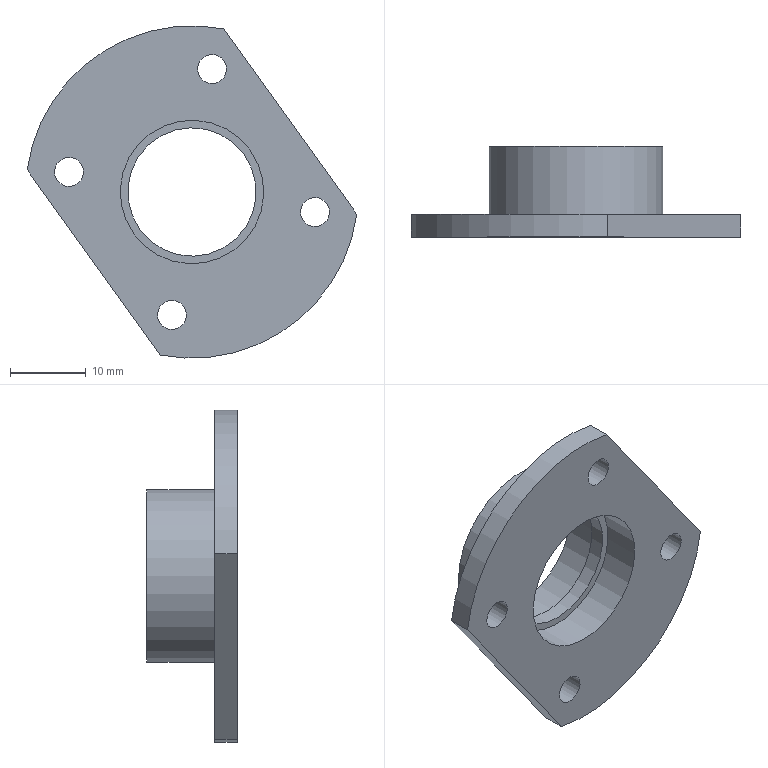Component | NX | BEARING_SLEEVE | 1 solid | 17 faces | volume 4126 mm3 | cylinder 10 | plane 7 | commonest cylinder face diameters 3.838 x4 44 x2 19 x2 17 x1 23 x1